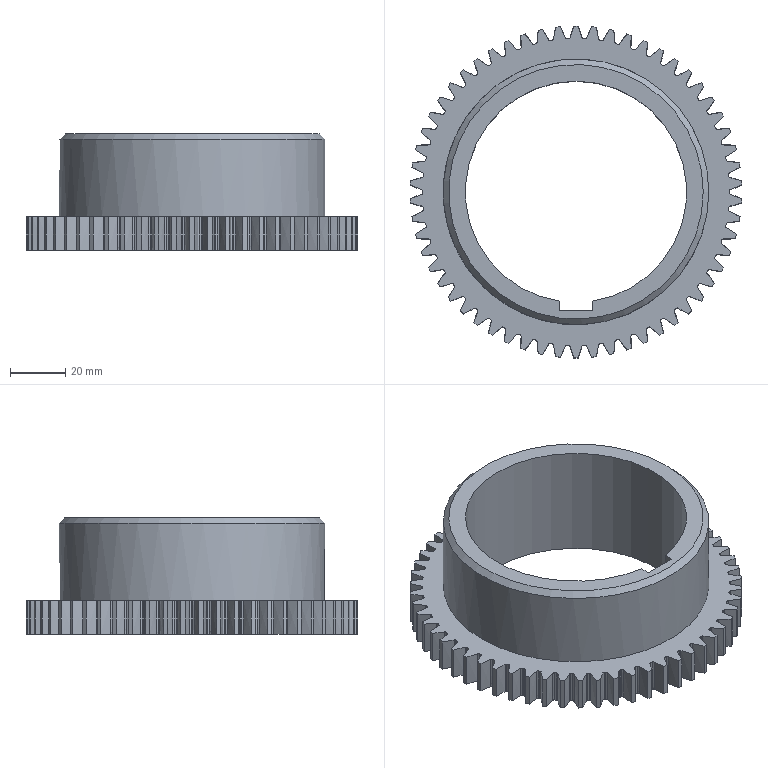Component | NX | CA6140-ZHUZHOU-CHILUN1 | 1 solid | 357 faces | volume 130054 mm3 | other 290 | cylinder 60 | plane 6 | cone 1 | commonest cylinder face diameters 111 x58 80 x1 96 x1